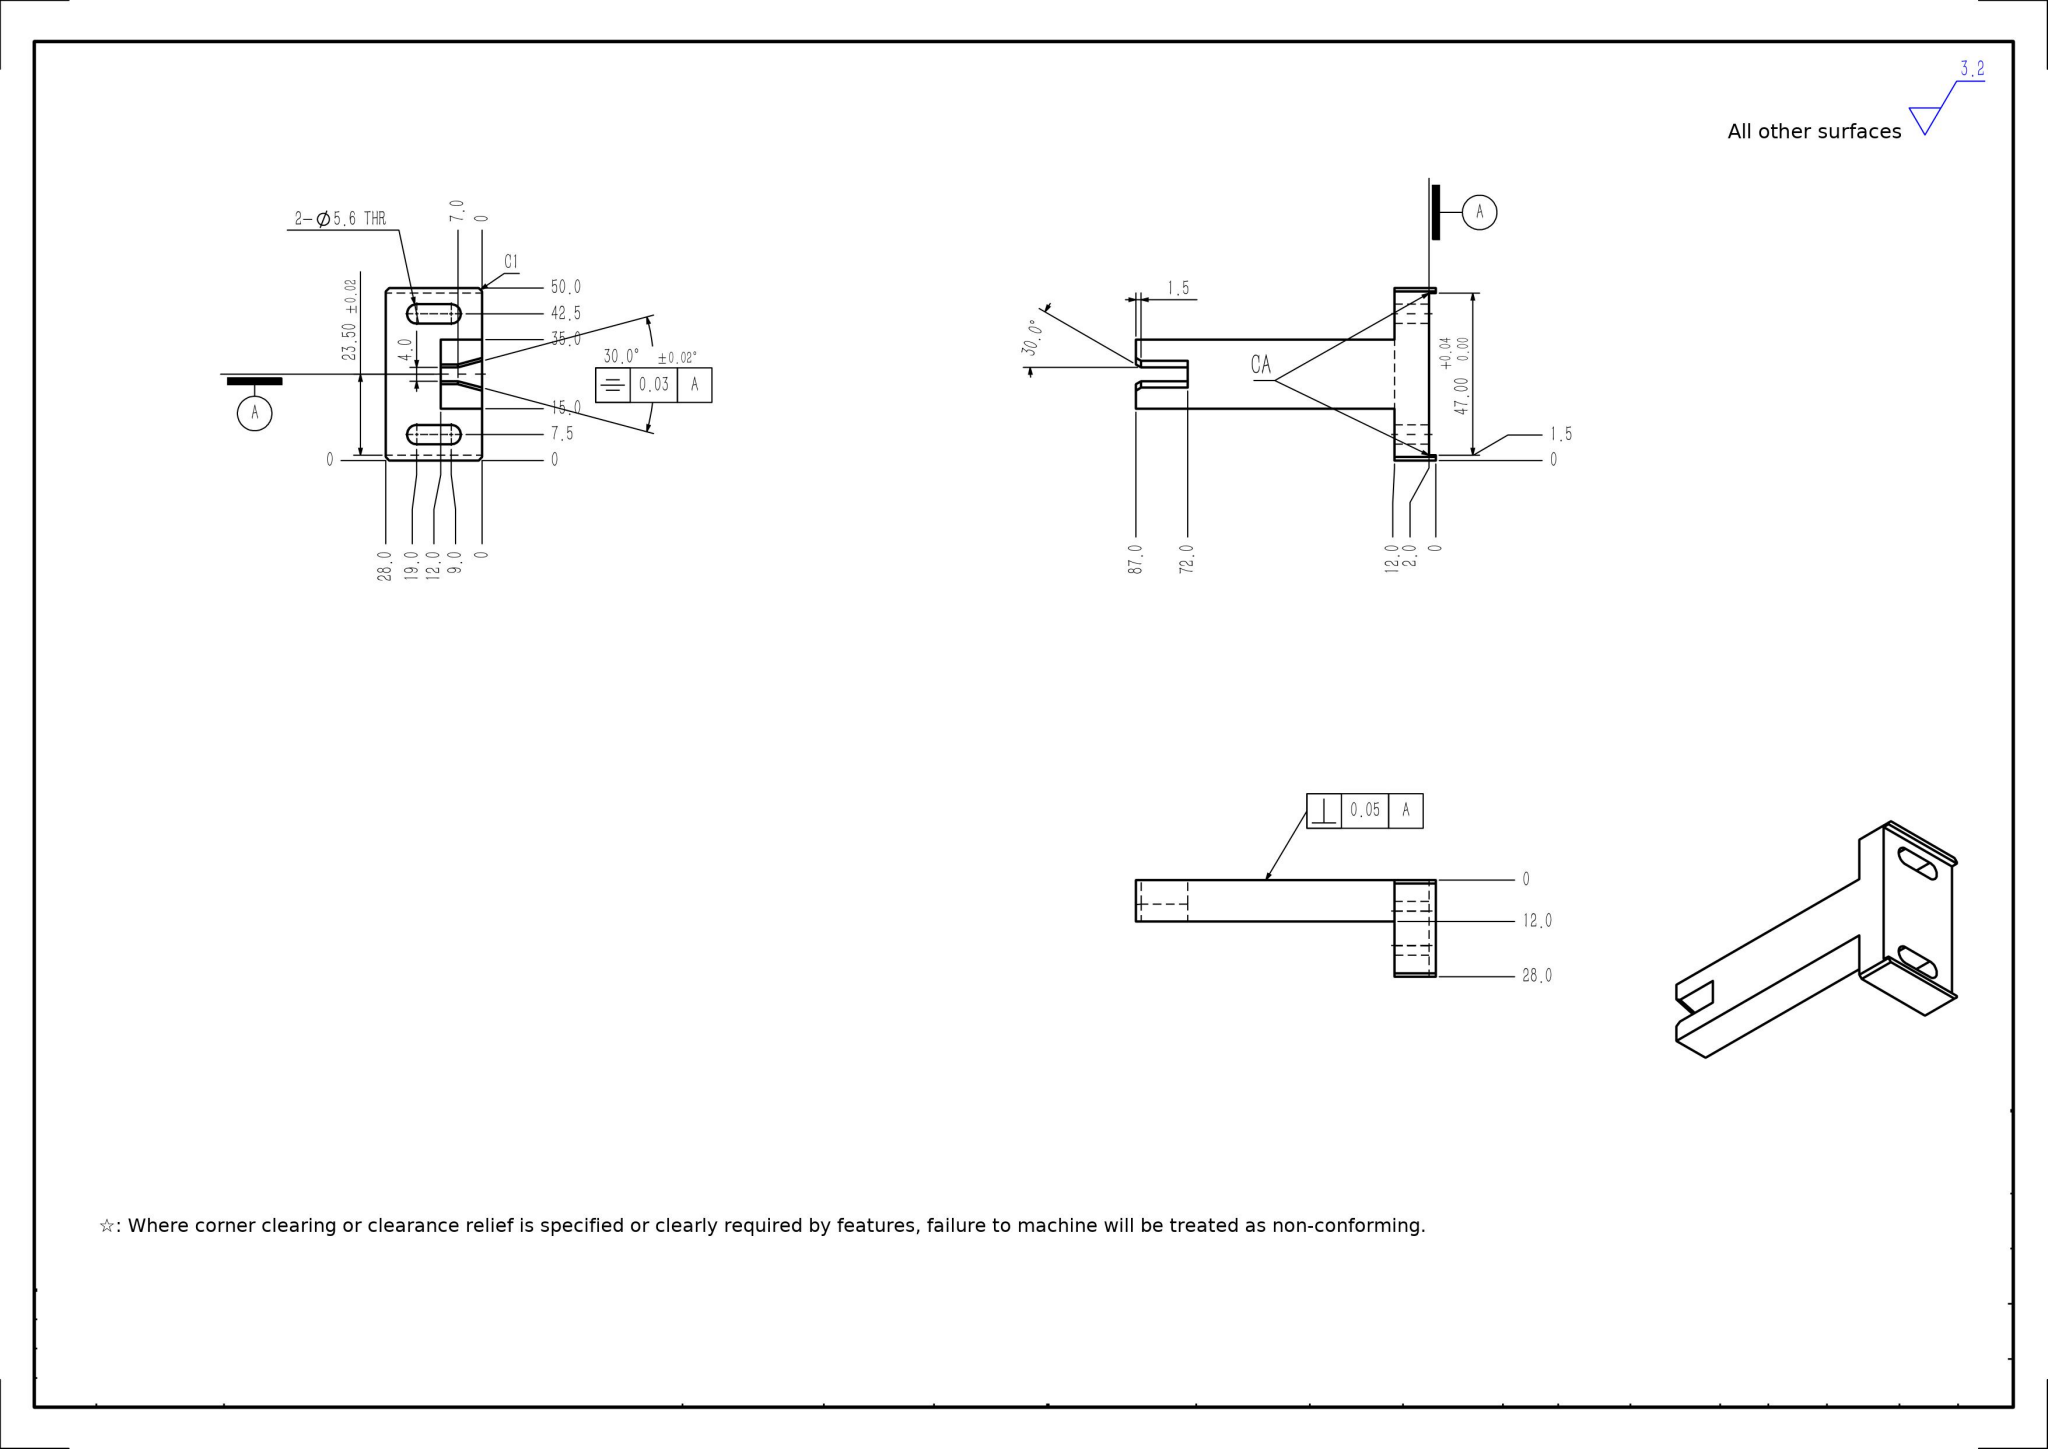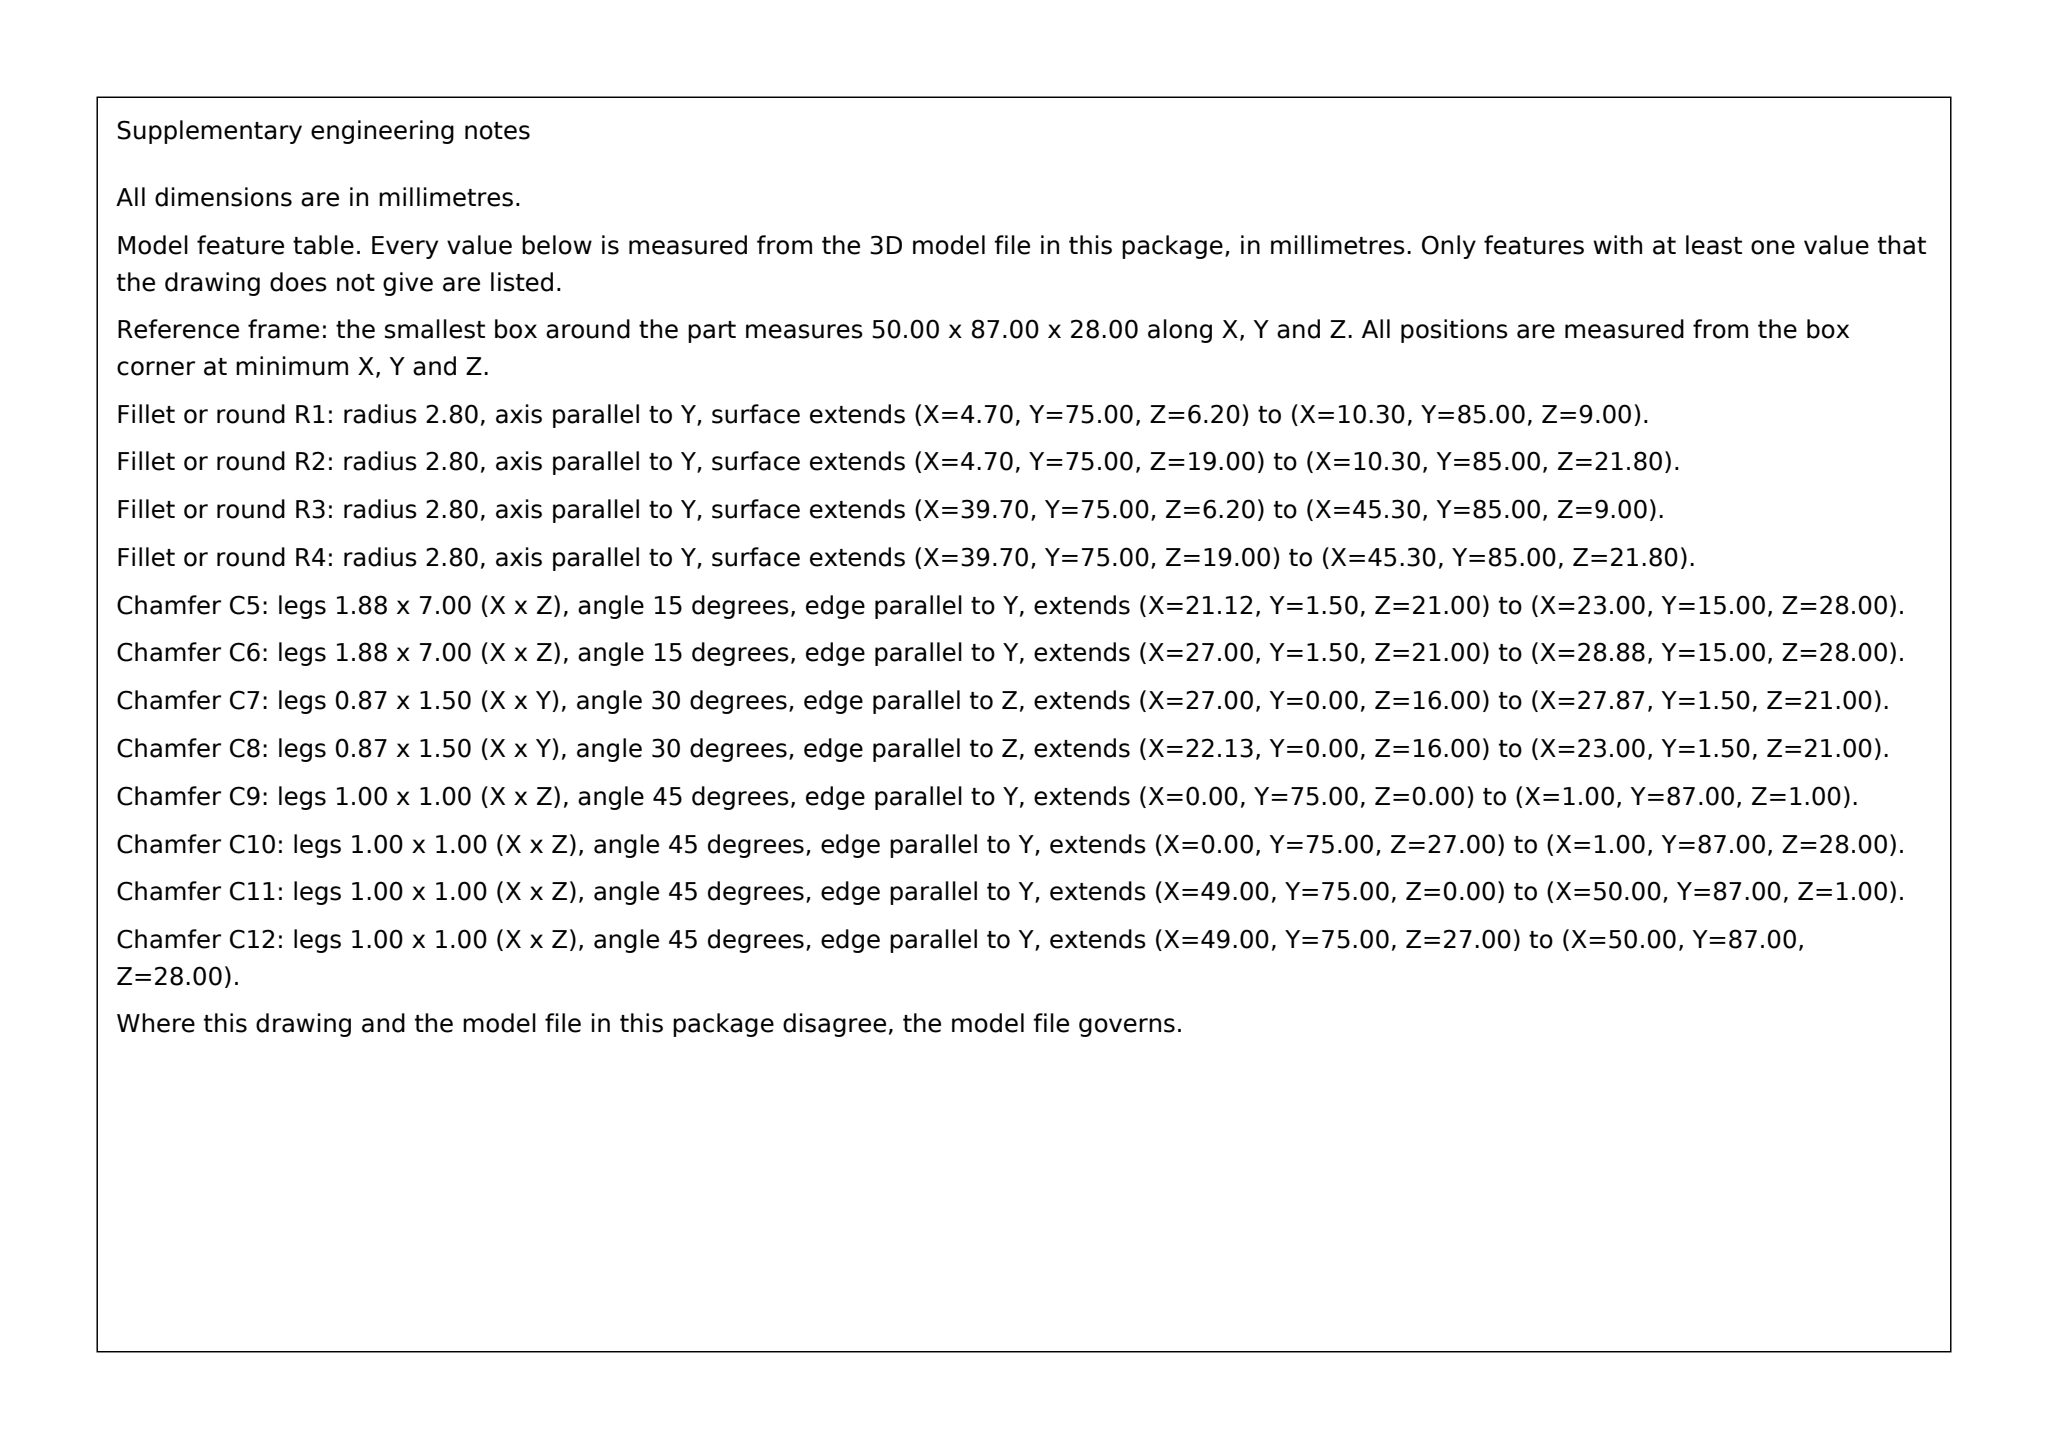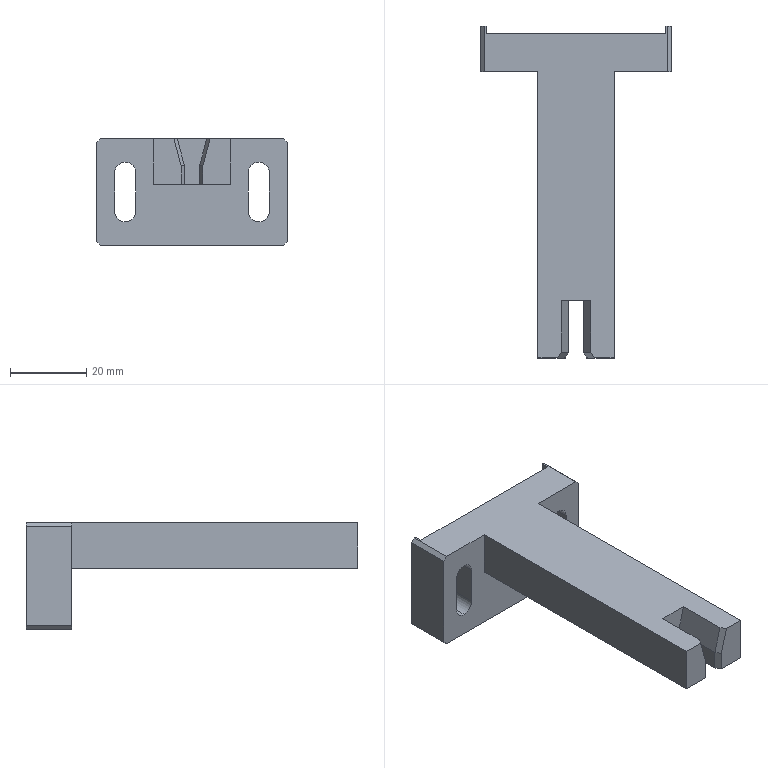Part | SolidWorks | mm | 1 solid | 38 faces | box 50 x 87 x 28 mm | volume 29599 mm3 | plane 32 | cylinder 6 | commonest cylinder face diameters 5.6 x6
build123d program:
from build123d import *
from OCP.BRepFilletAPI import BRepFilletAPI_MakeChamfer

# Parameters (mm, degrees)
BOSS_EXTRUDE1_DEPTH = 14
SKETCH2_W           = 16
SKETCH2_H           = 75
CUT_EXTRUDE1_DEPTH  = 58.561
CUT_EXTRUDE2_DEPTH  = 81.287
SKETCH5_W           = 4
SKETCH5_H           = 15
CUT_EXTRUDE4_DEPTH  = 53.662
CUT_EXTRUDE6_DEPTH  = 15
CHAMFER1_SIZE       = 1.5
CHAMFER1_SIZE2      = 0.866
CHAMFER2_SIZE       = 1
SKETCH10_W          = 47
SKETCH10_H          = 28
CUT_EXTRUDE7_DEPTH  = 2


with BuildPart() as part:
    # Sketch1 → Boss-Extrude1 (new, symmetric)
    with BuildSketch(Plane.XY):
        Polygon((-10, -43.5), (10, -43.5), (10, 31.5), (25, 31.5), (25, 43.5), (-25, 43.5), (-25, 31.5), (-10, 31.5), align=None)
    extrude(amount=BOSS_EXTRUDE1_DEPTH, both=True)

    # Sketch2 → Cut-Extrude1 (cut, through all)
    with BuildSketch(Plane(origin=(10, 0, 0), x_dir=(0, 0, -1), z_dir=(1, 0, 0))):
        with Locations((6, -6)):
            Rectangle(SKETCH2_W, SKETCH2_H)
    extrude(amount=-CUT_EXTRUDE1_DEPTH, mode=Mode.SUBTRACT)

    # Sketch3 → Cut-Extrude2 (cut, through all)
    with BuildSketch(Plane.XZ.offset(-31.5)):
        with BuildLine():
            Line((14.7, -5), (14.7, 5))
            ThreePointArc((14.7, 5), (17.5, 7.8), (20.3, 5))
            Line((20.3, 5), (20.3, -5))
            ThreePointArc((20.3, -5), (17.5, -7.8), (14.7, -5))
        make_face()
        with BuildLine():
            Line((-14.7, -5), (-14.7, 5))
            ThreePointArc((-14.7, 5), (-17.5, 7.8), (-20.3, 5))
            Line((-20.3, 5), (-20.3, -5))
            ThreePointArc((-20.3, -5), (-17.5, -7.8), (-14.7, -5))
        make_face()
    extrude(amount=-CUT_EXTRUDE2_DEPTH, mode=Mode.SUBTRACT)

    # Sketch5 → Cut-Extrude4 (cut, through all)
    with BuildSketch(Plane(origin=(0, 0, 2), x_dir=(-1, 0, 0), z_dir=(0, 0, -1))):
        with Locations((0, -36)):
            Rectangle(SKETCH5_W, SKETCH5_H)
    extrude(amount=-CUT_EXTRUDE4_DEPTH, mode=Mode.SUBTRACT)

    # Sketch9 → Cut-Extrude6 (cut)
    with BuildSketch(Plane(origin=(0, -43.5, 0), x_dir=(-1, 0, 0), z_dir=(0, -1, 0))):
        Polygon((3.876, -14), (-3.876, -14), (-2, -7), (2, -7), align=None)
    extrude(amount=-CUT_EXTRUDE6_DEPTH, mode=Mode.SUBTRACT)

    # Chamfer1: one chamfer whose edges measure the first distance from different faces: ONE call of the kernel's chamfer builder (chamfer() names one face for all edges)
    chamfer1_edges_1 = [part.edges().sort_by_distance(p)[0] for p in [
        (-2, -43.5, 4.5),
    ]]
    chamfer1_side_1 = [part.faces().sort_by_distance(p)[0] for p in [
        (-2, -36, 4.5),
    ]]
    chamfer1_edges_2 = [part.edges().sort_by_distance(p)[0] for p in [
        (2, -43.5, 4.5),
    ]]
    chamfer1_side_2 = [part.faces().sort_by_distance(p)[0] for p in [
        (2, -36, 4.5),
    ]]
    chamfer1_edges_3 = [part.edges().sort_by_distance(p)[0] for p in [
        (2.938, -43.5, 10.5),
    ]]
    chamfer1_side_3 = [part.faces().sort_by_distance(p)[0] for p in [
        (2.938, -36, 10.5),
    ]]
    chamfer1_edges_4 = [part.edges().sort_by_distance(p)[0] for p in [
        (-2.938, -43.5, 10.5),
    ]]
    chamfer1_side_4 = [part.faces().sort_by_distance(p)[0] for p in [
        (-2.938, -36, 10.5),
    ]]
    chamfer1 = BRepFilletAPI_MakeChamfer(part.part.solid().wrapped)
    for e in chamfer1_edges_1:
        chamfer1.Add(CHAMFER1_SIZE, CHAMFER1_SIZE2, e.wrapped, chamfer1_side_1[0].wrapped)  # the first distance lies on this face
    for e in chamfer1_edges_2:
        chamfer1.Add(CHAMFER1_SIZE, CHAMFER1_SIZE2, e.wrapped, chamfer1_side_2[0].wrapped)  # the first distance lies on this face
    for e in chamfer1_edges_3:
        chamfer1.Add(CHAMFER1_SIZE, CHAMFER1_SIZE2, e.wrapped, chamfer1_side_3[0].wrapped)  # the first distance lies on this face
    for e in chamfer1_edges_4:
        chamfer1.Add(CHAMFER1_SIZE, CHAMFER1_SIZE2, e.wrapped, chamfer1_side_4[0].wrapped)  # the first distance lies on this face
    add(Compound.cast(chamfer1.Shape()), mode=Mode.REPLACE)

    # Chamfer2
    chamfer2_edges = [part.edges().sort_by_distance(p)[0] for p in [
        (-25, 37.5, 14),
        (25, 37.5, -14),
        (25, 37.5, 14),
        (-25, 37.5, -14),
    ]]
    chamfer(chamfer2_edges, length=CHAMFER2_SIZE)

    # Sketch10 → Cut-Extrude7 (cut)
    with BuildSketch(Plane(origin=(0, 43.5, 0), x_dir=(1, 0, 0), z_dir=(0, 1, 0))):
        Rectangle(SKETCH10_W, SKETCH10_H)
    extrude(amount=-CUT_EXTRUDE7_DEPTH, mode=Mode.SUBTRACT)


solid = part.part